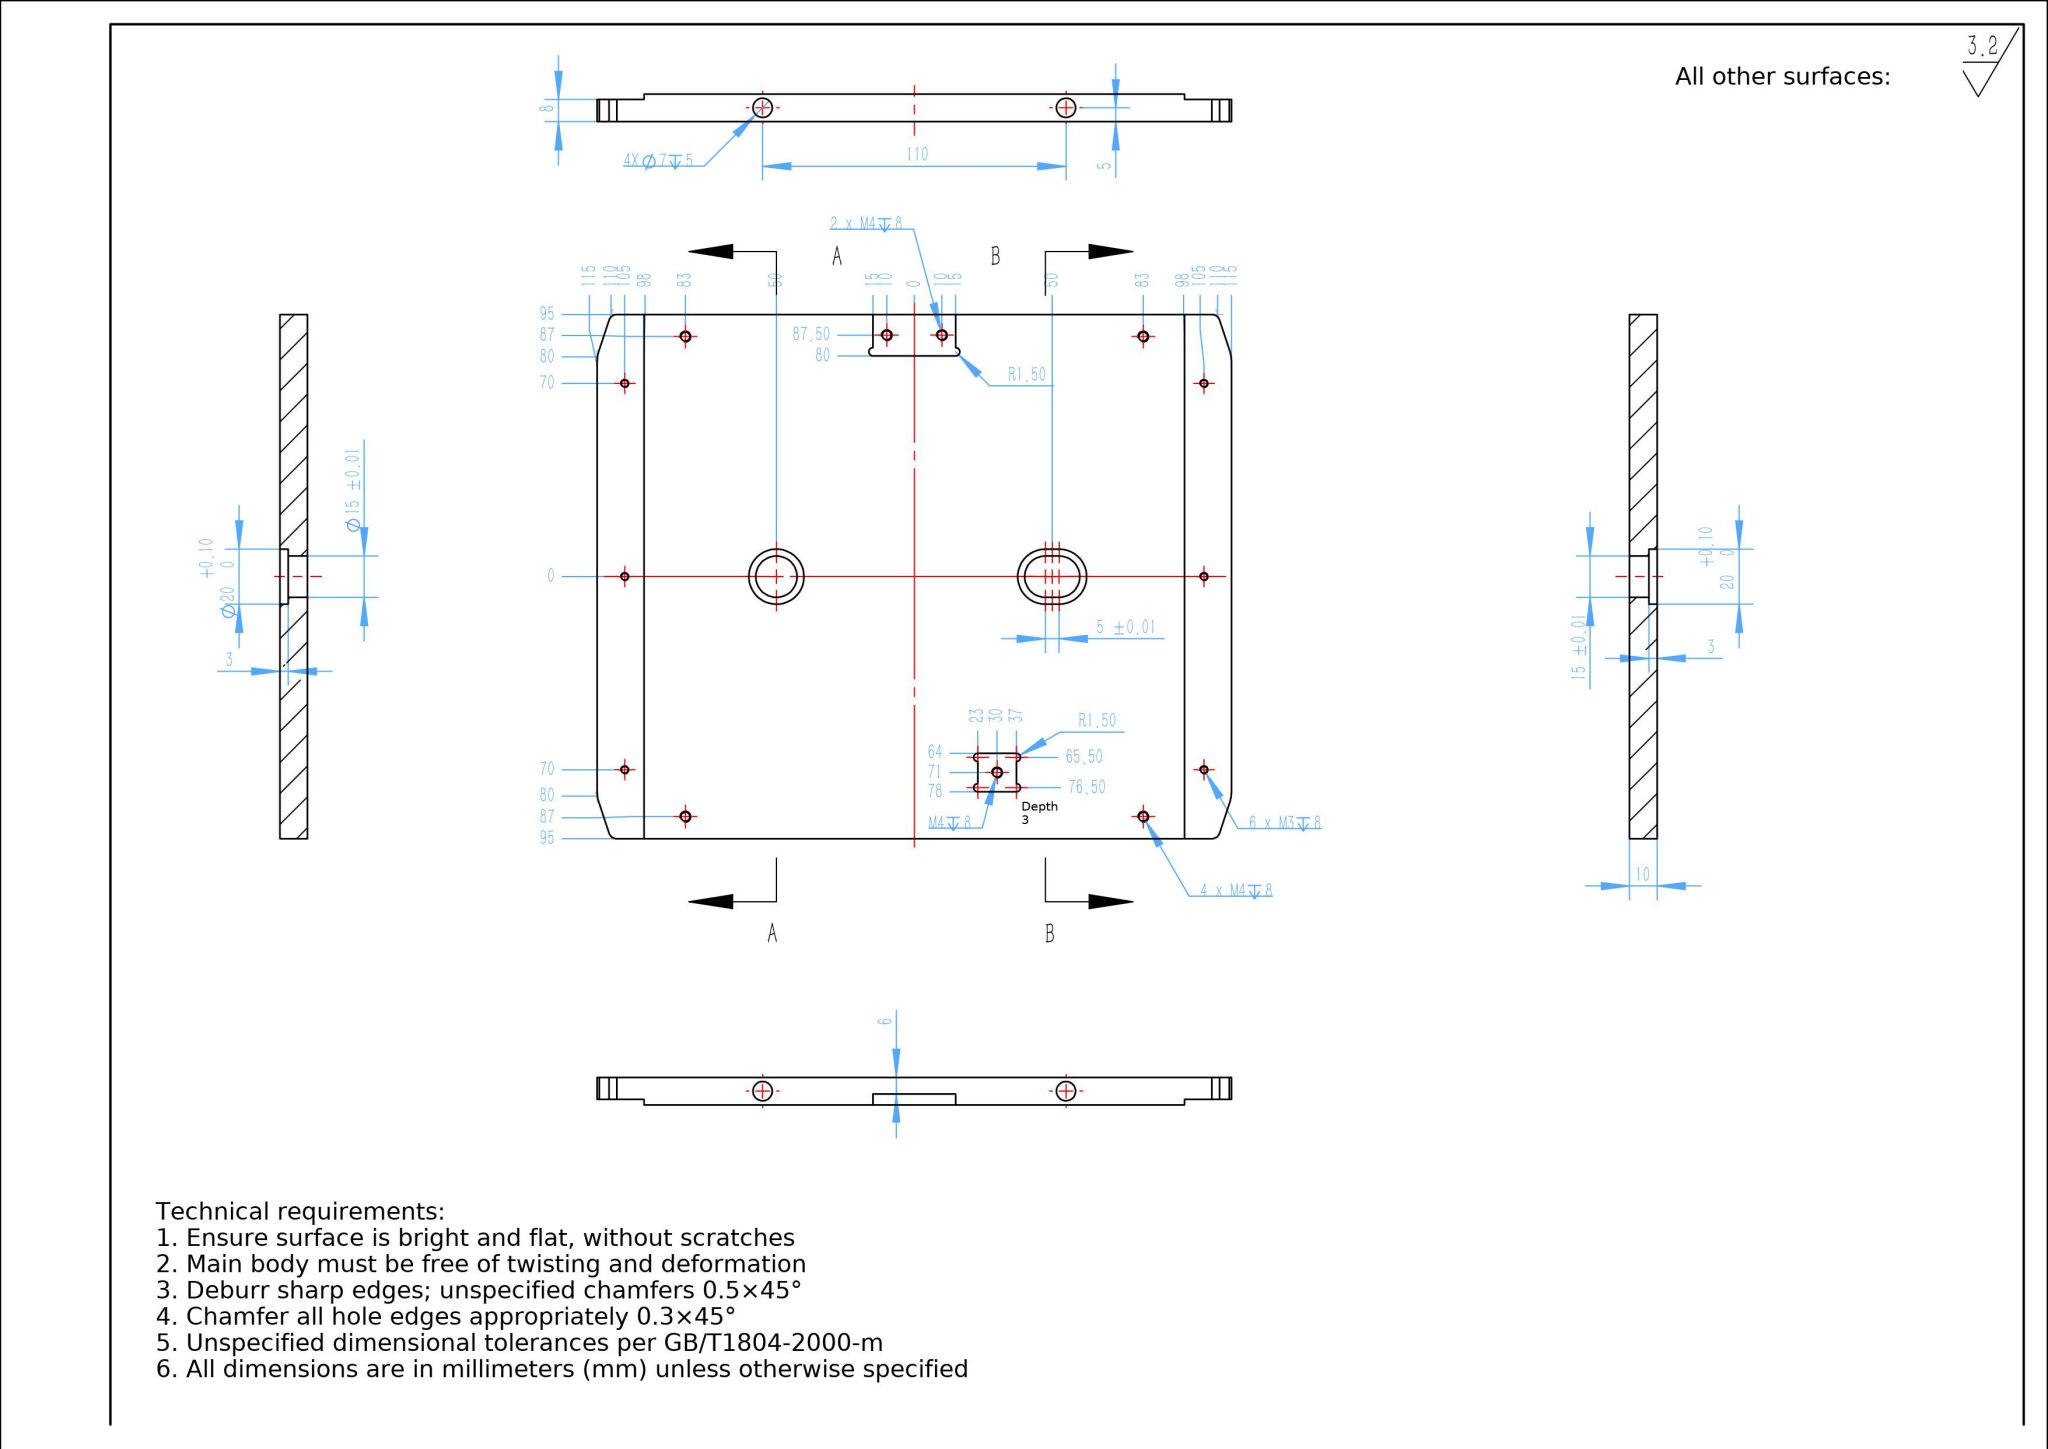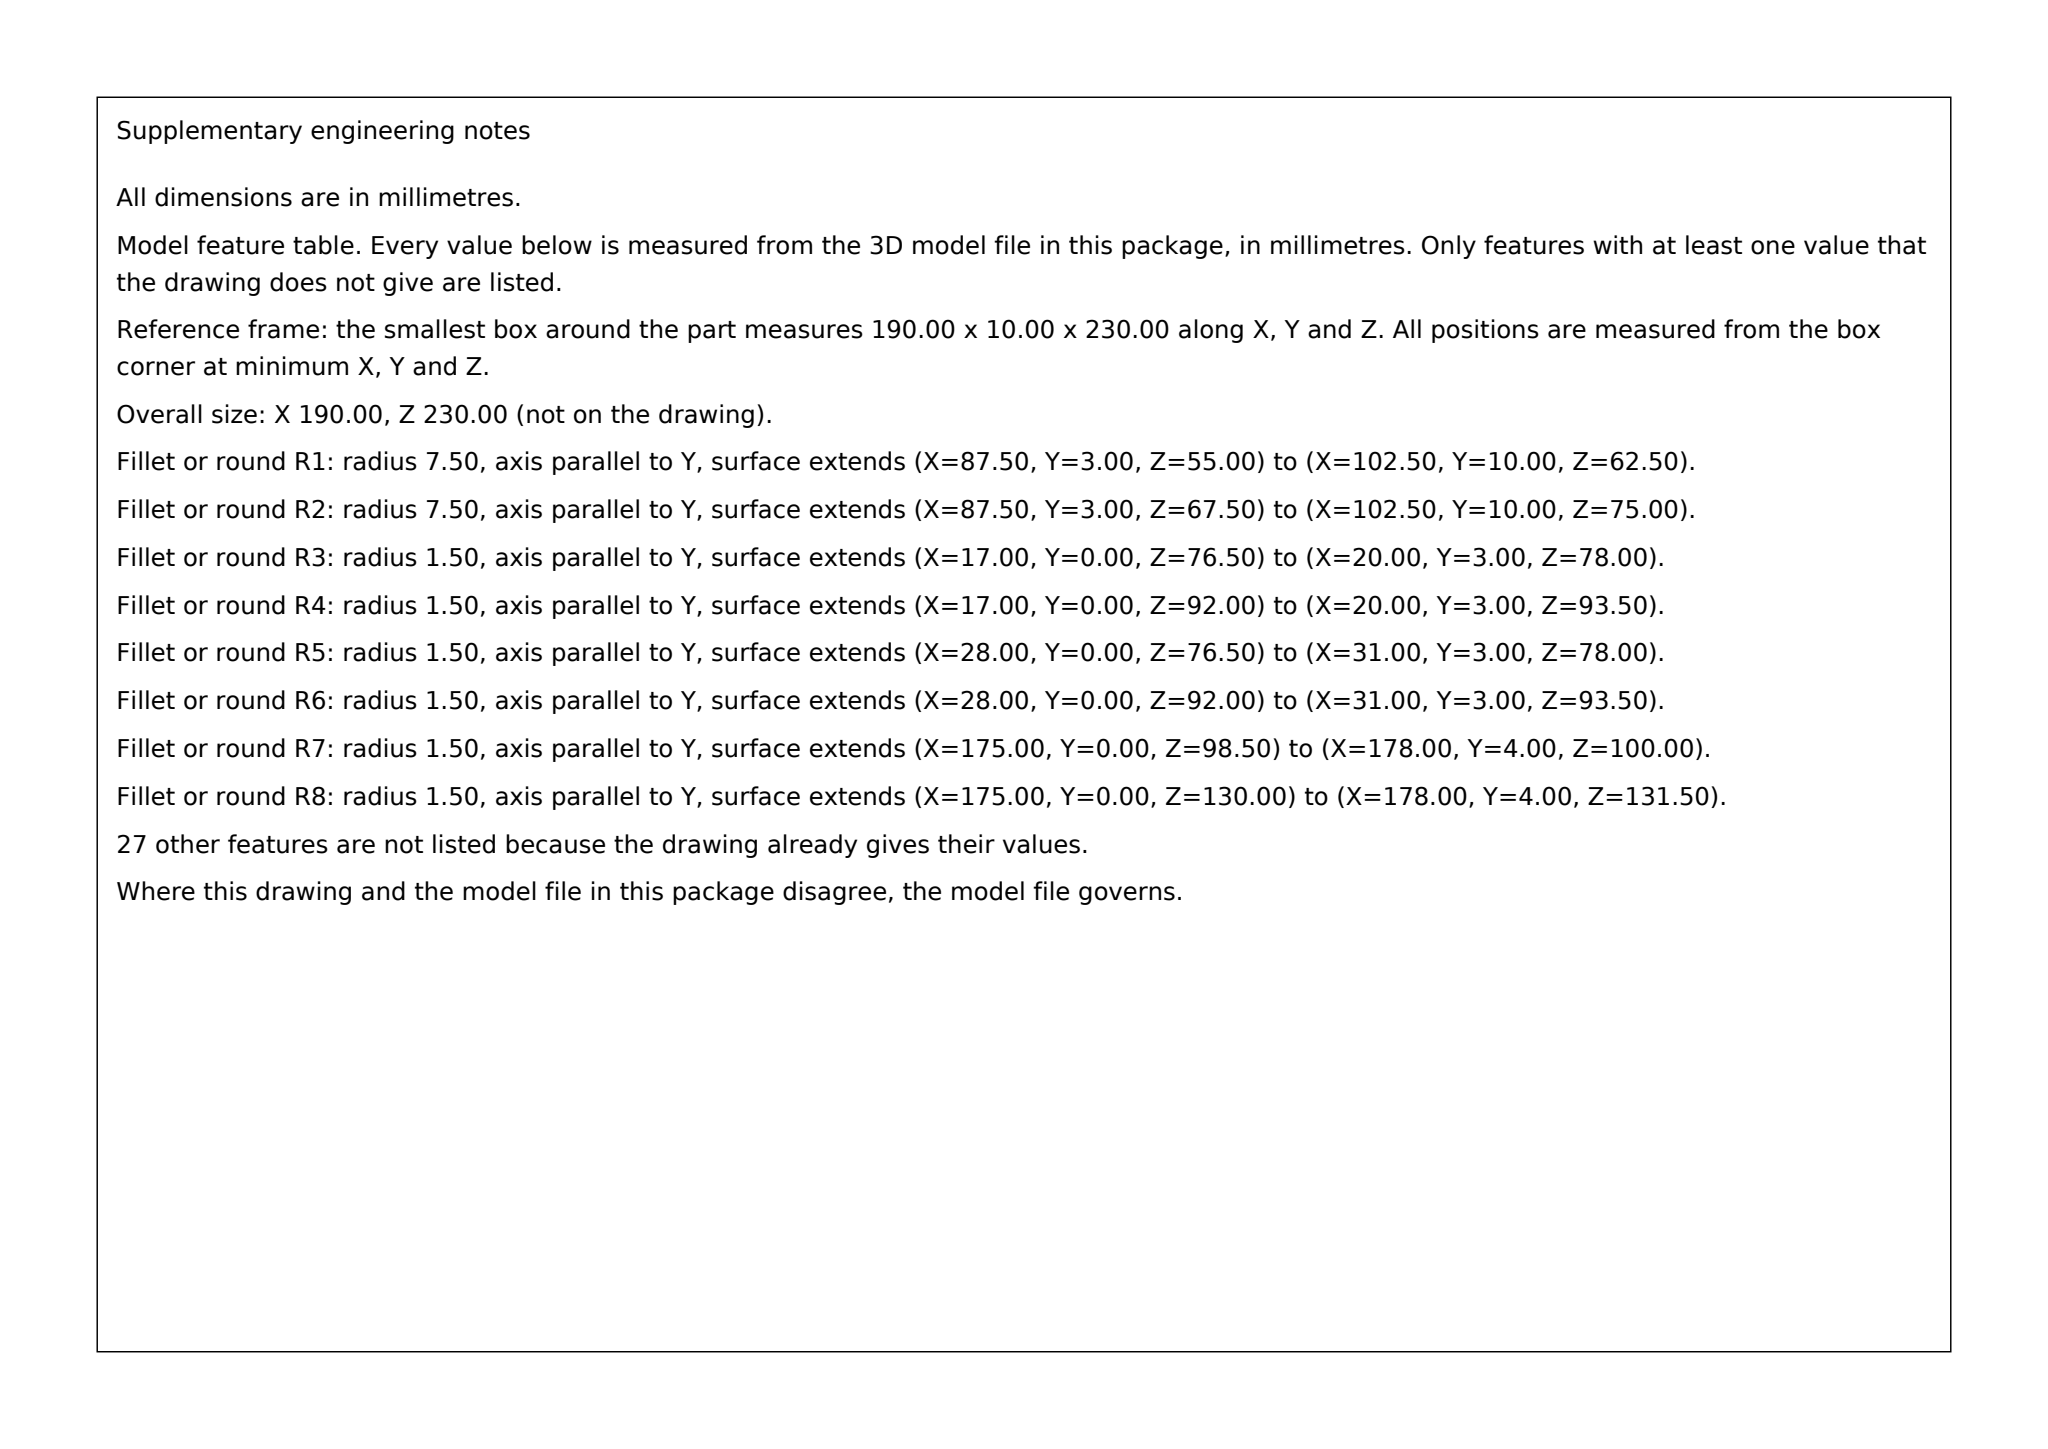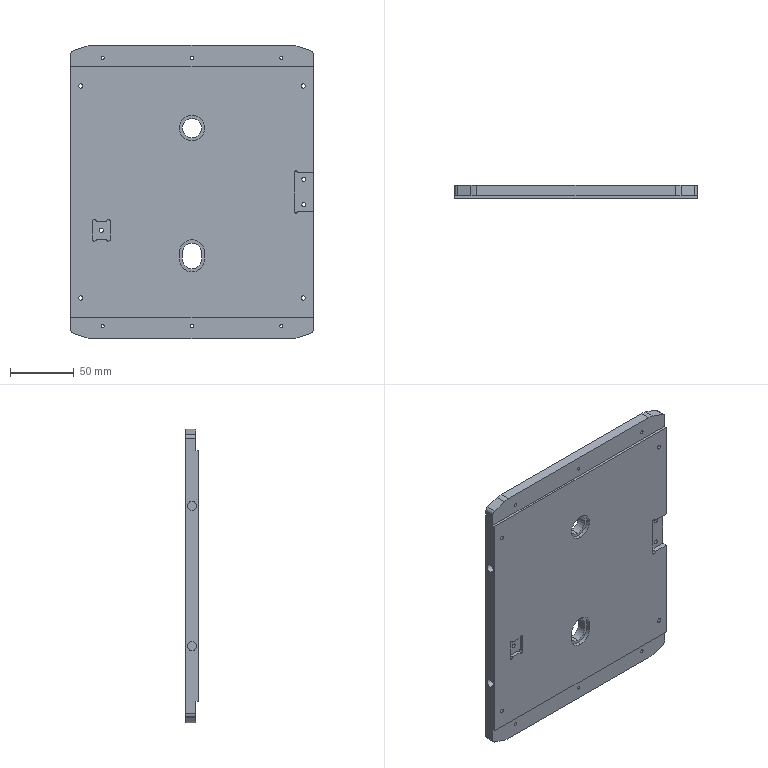Part | SolidWorks | mm | 1 solid | 94 faces | box 190 x 10 x 230 mm | volume 413690 mm3 | cylinder 61 | plane 33 | commonest cylinder face diameters 3.3 x14 2.5 x12 3 x9 7 x8 15 x5 20 x5 30 x4 6 x4
build123d program:
from build123d import *

# Parameters (mm, degrees)
SKETCH1_W             = 190
SKETCH1_H             = 230
BOSS_EXTRUDE1_DEPTH   = 10
CUT_EXTRUDE1_DEPTH    = 150.499
FILLET1_R             = 15
FILLET2_R             = 3
SKETCH3_OUTSIDE_W     = 251.7
SKETCH3_OUTSIDE_H     = 291.7
SKETCH3_OUTSIDE_W_2   = 190
SKETCH3_OUTSIDE_H_2   = 196
CUT_EXTRUDE2_DEPTH    = 2
M3_TAPPED_HOLE1_D     = 2.5
M3_TAPPED_HOLE1_DEPTH = 9
M3_TAPPED_HOLE1_TIP   = 0.7511
SKETCH6_R             = 10
CUT_EXTRUDE3_DEPTH    = 3
SKETCH7_R             = 7.5
CUT_EXTRUDE4_DEPTH    = 150.328
M4_TAPPED_HOLE1_D     = 3.3
M4_TAPPED_HOLE1_DEPTH = 10.1
M4_TAPPED_HOLE1_TIP   = 0.9914
SKETCH11_W            = 15
SKETCH11_H            = 30
CUT_EXTRUDE5_DEPTH    = 4
CUT_EXTRUDE6_DEPTH    = 4
M4_TAPPED_HOLE2_D     = 3.3
M4_TAPPED_HOLE2_DEPTH = 10.1
M4_TAPPED_HOLE2_TIP   = 0.9914
SKETCH15_W            = 14
SKETCH15_H            = 14
CUT_EXTRUDE7_DEPTH    = 3
CUT_EXTRUDE8_DEPTH    = 3
M4_TAPPED_HOLE3_D     = 3.3
M4_TAPPED_HOLE3_DEPTH = 10.1
M4_TAPPED_HOLE3_TIP   = 0.9914
SKETCH19_R            = 3.5
CUT_EXTRUDE9_DEPTH    = 5


with BuildPart() as part:
    # Sketch1 → Boss-Extrude1 (new body)
    with BuildSketch(Plane(origin=(0, 0, 0), x_dir=(1, 0, 0), z_dir=(0, 1, 0))):
        Rectangle(SKETCH1_W, SKETCH1_H)
    extrude(amount=BOSS_EXTRUDE1_DEPTH)

    # Sketch2 → Cut-Extrude1 (cut, through all)
    with BuildSketch(Plane(origin=(0, 10, 0), x_dir=(1, 0, 0), z_dir=(0, 1, 0))):
        Polygon((-80, 115), (-95, 110), (-95, 115), align=None)
        Polygon((95, 115), (95, 110), (80, 115), align=None)
        Polygon((80, -115), (95, -110), (95, -115), align=None)
        Polygon((-95, -115), (-95, -110), (-80, -115), align=None)
    extrude(amount=-CUT_EXTRUDE1_DEPTH, mode=Mode.SUBTRACT)

    # Fillet1
    fillet1_edges = [part.edges().sort_by_distance(p)[0] for p in [
        (-80, 5, -115),
        (80, 5, -115),
        (80, 5, 115),
        (-80, 5, 115),
    ]]
    fillet(fillet1_edges, radius=FILLET1_R)

    # Fillet2
    fillet2_edges = [part.edges().sort_by_distance(p)[0] for p in [
        (-95, 5, -110),
        (95, 5, -110),
        (95, 5, 110),
        (-95, 5, 110),
    ]]
    fillet(fillet2_edges, radius=FILLET2_R)

    # Sketch3 outside → Cut-Extrude2 (cut)
    with BuildSketch(Plane.XZ):
        Rectangle(SKETCH3_OUTSIDE_W, SKETCH3_OUTSIDE_H)
        Rectangle(SKETCH3_OUTSIDE_W_2, SKETCH3_OUTSIDE_H_2, mode=Mode.SUBTRACT)
    extrude(amount=-CUT_EXTRUDE2_DEPTH, mode=Mode.SUBTRACT)

    # M3 Tapped Hole1
    with Locations(Plane(origin=(0, 2, 0), x_dir=(-1, 0, 0), z_dir=(0, -1, 0))):
        with Locations((70, -105), (-70, -105), (0, -105), (0, 105), (-70, 105), (70, 105)):
            Hole(M3_TAPPED_HOLE1_D / 2, depth=M3_TAPPED_HOLE1_DEPTH)
            with Locations((0, 0, -(M3_TAPPED_HOLE1_DEPTH + M3_TAPPED_HOLE1_TIP / 2))):  # 118° drill point
                Cone(0, M3_TAPPED_HOLE1_D / 2, M3_TAPPED_HOLE1_TIP, mode=Mode.SUBTRACT)

    # Sketch6 → Cut-Extrude3 (cut)
    with BuildSketch(Plane.XZ):
        with Locations(Location((0, 50, 0), (0, 0, 270))):
            Circle(SKETCH6_R)
        with BuildLine():
            Line((-10, -52.5), (-10, -47.5))
            ThreePointArc((-10, -47.5), (0, -37.5), (10, -47.5))
            Line((10, -47.5), (10, -52.5))
            ThreePointArc((10, -52.5), (0, -62.5), (-10, -52.5))
        make_face()
    extrude(amount=-CUT_EXTRUDE3_DEPTH, mode=Mode.SUBTRACT)

    # Sketch7 → Cut-Extrude4 (cut, through all)
    with BuildSketch(Plane.XZ.offset(-3)):
        with Locations(Location((0, 50, 0), (0, 0, 270))):
            Circle(SKETCH7_R)
        with BuildLine():
            Line((7.5, -52.5), (7.5, -47.5))
            ThreePointArc((7.5, -47.5), (0, -40), (-7.5, -47.5))
            Line((-7.5, -47.5), (-7.5, -52.5))
            ThreePointArc((-7.5, -52.5), (0, -60), (7.5, -52.5))
        make_face()
    extrude(amount=-CUT_EXTRUDE4_DEPTH, mode=Mode.SUBTRACT)

    # M4 Tapped Hole1
    with Locations(Plane(origin=(0, 10, 0), x_dir=(1, 0, 0), z_dir=(0, 1, 0))):
        with Locations((-87, -83), (87, -83), (87, 83), (-87, 83)):
            Hole(M4_TAPPED_HOLE1_D / 2, depth=M4_TAPPED_HOLE1_DEPTH)
            with Locations((0, 0, -(M4_TAPPED_HOLE1_DEPTH + M4_TAPPED_HOLE1_TIP / 2))):  # 118° drill point
                Cone(0, M4_TAPPED_HOLE1_D / 2, M4_TAPPED_HOLE1_TIP, mode=Mode.SUBTRACT)

    # Sketch11 → Cut-Extrude5 (cut)
    with BuildSketch(Plane.XZ):
        with Locations((87.5, 0)):
            Rectangle(SKETCH11_W, SKETCH11_H)
    extrude(amount=-CUT_EXTRUDE5_DEPTH, mode=Mode.SUBTRACT)

    # Sketch12 → Cut-Extrude6 (cut)
    with BuildSketch(Plane.XZ):
        with BuildLine():
            Line((80, 15), (83, 15))
            ThreePointArc((83, 15), (81.5, 16.5), (80, 15))
        make_face()
        with BuildLine():
            Line((80, -15), (83, -15))
            ThreePointArc((83, -15), (81.5, -16.5), (80, -15))
        make_face()
    extrude(amount=-CUT_EXTRUDE6_DEPTH, mode=Mode.SUBTRACT)

    # M4 Tapped Hole2
    with Locations(Plane(origin=(0, 4, 0), x_dir=(-1, 0, 0), z_dir=(0, -1, 0))):
        with Locations((-87.5, -10), (-87.5, 10)):
            Hole(M4_TAPPED_HOLE2_D / 2, depth=M4_TAPPED_HOLE2_DEPTH)
            with Locations((0, 0, -(M4_TAPPED_HOLE2_DEPTH + M4_TAPPED_HOLE2_TIP / 2))):  # 118° drill point
                Cone(0, M4_TAPPED_HOLE2_D / 2, M4_TAPPED_HOLE2_TIP, mode=Mode.SUBTRACT)

    # Sketch15 → Cut-Extrude7 (cut)
    with BuildSketch(Plane.XZ):
        with Locations((-71, -30)):
            Rectangle(SKETCH15_W, SKETCH15_H)
    extrude(amount=-CUT_EXTRUDE7_DEPTH, mode=Mode.SUBTRACT)

    # Sketch16 → Cut-Extrude8 (cut)
    with BuildSketch(Plane.XZ):
        with BuildLine():
            Line((-78, -23), (-75, -23))
            ThreePointArc((-75, -23), (-76.5, -21.5), (-78, -23))
        make_face()
        with BuildLine():
            Line((-64, -23), (-67, -23))
            ThreePointArc((-67, -23), (-65.5, -21.5), (-64, -23))
        make_face()
        with BuildLine():
            Line((-78, -37), (-75, -37))
            ThreePointArc((-75, -37), (-76.5, -38.5), (-78, -37))
        make_face()
        with BuildLine():
            Line((-67, -37), (-64, -37))
            ThreePointArc((-64, -37), (-65.5, -38.5), (-67, -37))
        make_face()
    extrude(amount=-CUT_EXTRUDE8_DEPTH, mode=Mode.SUBTRACT)

    # M4 Tapped Hole3
    with Locations(Plane(origin=(0, 3, 0), x_dir=(-1, 0, 0), z_dir=(0, -1, 0))):
        with Locations((71, 30)):
            Hole(M4_TAPPED_HOLE3_D / 2, depth=M4_TAPPED_HOLE3_DEPTH)
            with Locations((0, 0, -(M4_TAPPED_HOLE3_DEPTH + M4_TAPPED_HOLE3_TIP / 2))):  # 118° drill point
                Cone(0, M4_TAPPED_HOLE3_D / 2, M4_TAPPED_HOLE3_TIP, mode=Mode.SUBTRACT)

    # Sketch19 → Cut-Extrude9 (cut)
    with BuildSketch(Plane(origin=(95, 0, 0), x_dir=(0, 0, -1), z_dir=(1, 0, 0))):
        with Locations((-55, 5)):
            Circle(SKETCH19_R)
        with Locations(Location((55, 5, 0), (0, 0, 180))):
            Circle(SKETCH19_R)
    cut_extrude9 = extrude(amount=-CUT_EXTRUDE9_DEPTH, mode=Mode.SUBTRACT)

    # Mirror1: Cut-Extrude9 across plane
    add(cut_extrude9.mirror(Plane(origin=(0, 0, 0), x_dir=(0, 0, 1), z_dir=(1, 0, 0))), mode=Mode.SUBTRACT)


solid = part.part